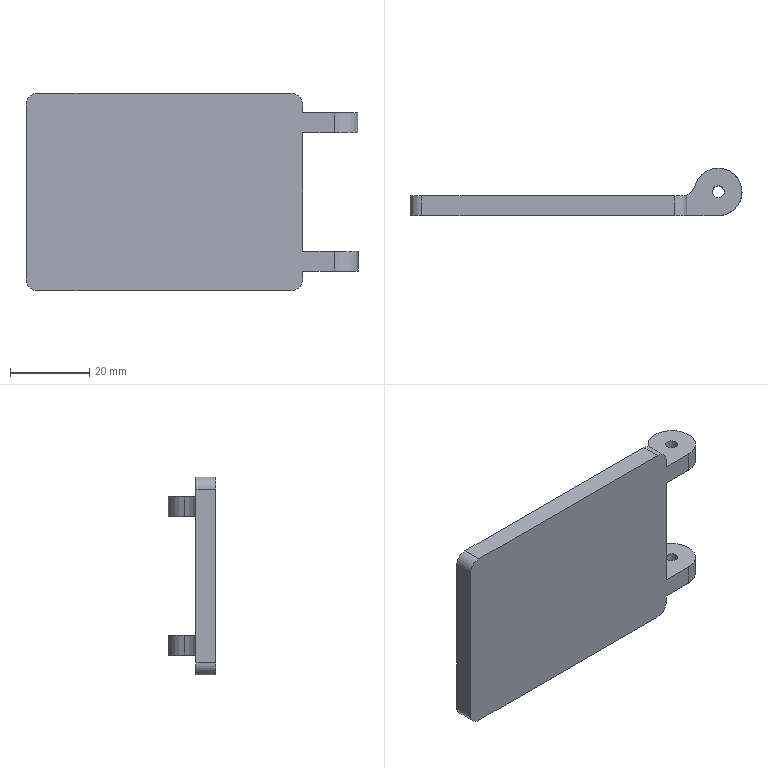Component | SolidWorks | 22FuelTankCap-1 | 1 solid | 25 faces | box 84 x 12 x 50 mm | volume 18718 mm3 | cylinder 13 | plane 12 | commonest cylinder face diameters 12 x5 3 x4 6 x4
STEP:
#1=CARTESIAN_POINT('',(3.204,14.835,19.37));
#2=VERTEX_POINT('',#1);
#3=CARTESIAN_POINT('',(3.322,14.835,19.37));
#4=VERTEX_POINT('',#3);
#5=CARTESIAN_POINT('',(3.263,14.835,19.37));
#6=DIRECTION('',(0.,0.,1.));
#7=DIRECTION('',(1.,0.,0.));
#8=AXIS2_PLACEMENT_3D('',#5,#6,#7);
#9=CIRCLE('',#8,0.05906);
#10=EDGE_CURVE('',#2,#4,#9,.T.);
#11=ORIENTED_EDGE('',*,*,#10,.F.);
#12=CARTESIAN_POINT('',(3.204,14.835,19.567));
#13=VERTEX_POINT('',#12);
#14=CARTESIAN_POINT('',(3.204,14.835,19.37));
#15=DIRECTION('',(0.,0.,1.));
#16=VECTOR('',#15,39.37);
#17=LINE('',#14,#16);
#18=EDGE_CURVE('',#2,#13,#17,.T.);
#19=ORIENTED_EDGE('',*,*,#18,.T.);
#20=CARTESIAN_POINT('',(3.322,14.835,19.567));
#21=VERTEX_POINT('',#20);
#22=CARTESIAN_POINT('',(3.263,14.835,19.567));
#23=DIRECTION('',(0.,0.,1.));
#24=DIRECTION('',(1.,0.,0.));
#25=AXIS2_PLACEMENT_3D('',#22,#23,#24);
#26=CIRCLE('',#25,0.05906);
#27=EDGE_CURVE('',#13,#21,#26,.T.);
#28=ORIENTED_EDGE('',*,*,#27,.T.);
#29=CARTESIAN_POINT('',(3.322,14.835,19.37));
#30=DIRECTION('',(0.,0.,1.));
#31=VECTOR('',#30,39.37);
#32=LINE('',#29,#31);
#33=EDGE_CURVE('',#4,#21,#32,.T.);
#34=ORIENTED_EDGE('',*,*,#33,.F.);
#35=EDGE_LOOP('',(#11,#19,#28,#34));
#36=FACE_OUTER_BOUND('',#35,.T.);
#37=CARTESIAN_POINT('',(3.263,14.835,19.37));
#38=DIRECTION('',(0.,0.,1.));
#39=DIRECTION('',(1.,0.,0.));
#40=AXIS2_PLACEMENT_3D('',#37,#38,#39);
#41=CYLINDRICAL_SURFACE('',#40,0.05906);
#42=ADVANCED_FACE('',(#36),#41,.F.);
#43=CARTESIAN_POINT('',(3.263,14.599,19.37));
#44=VERTEX_POINT('',#43);
#45=CARTESIAN_POINT('',(3.499,14.835,19.37));
#46=VERTEX_POINT('',#45);
#47=CARTESIAN_POINT('',(3.263,14.835,19.37));
#48=DIRECTION('',(0.,0.,1.));
#49=DIRECTION('',(1.,0.,0.));
#50=AXIS2_PLACEMENT_3D('',#47,#48,#49);
#51=CIRCLE('',#50,0.2362);
#52=EDGE_CURVE('',#44,#46,#51,.T.);
#53=ORIENTED_EDGE('',*,*,#52,.T.);
#54=CARTESIAN_POINT('',(3.499,14.835,19.567));
#55=VERTEX_POINT('',#54);
#56=CARTESIAN_POINT('',(3.499,14.835,19.37));
#57=DIRECTION('',(0.,0.,1.));
#58=VECTOR('',#57,39.37);
#59=LINE('',#56,#58);
#60=EDGE_CURVE('',#46,#55,#59,.T.);
#61=ORIENTED_EDGE('',*,*,#60,.T.);
#62=CARTESIAN_POINT('',(3.263,14.599,19.567));
#63=VERTEX_POINT('',#62);
#64=CARTESIAN_POINT('',(3.263,14.835,19.567));
#65=DIRECTION('',(0.,0.,1.));
#66=DIRECTION('',(1.,0.,0.));
#67=AXIS2_PLACEMENT_3D('',#64,#65,#66);
#68=CIRCLE('',#67,0.2362);
#69=EDGE_CURVE('',#63,#55,#68,.T.);
#70=ORIENTED_EDGE('',*,*,#69,.F.);
#71=CARTESIAN_POINT('',(3.263,14.599,19.37));
#72=DIRECTION('',(0.,0.,1.));
#73=VECTOR('',#72,39.37);
#74=LINE('',#71,#73);
#75=EDGE_CURVE('',#44,#63,#74,.T.);
#76=ORIENTED_EDGE('',*,*,#75,.F.);
#77=EDGE_LOOP('',(#53,#61,#70,#76));
#78=FACE_OUTER_BOUND('',#77,.T.);
#79=CARTESIAN_POINT('',(3.263,14.835,19.37));
#80=DIRECTION('',(0.,0.,1.));
#81=DIRECTION('',(1.,0.,0.));
#82=AXIS2_PLACEMENT_3D('',#79,#80,#81);
#83=CYLINDRICAL_SURFACE('',#82,0.2362);
#84=ADVANCED_FACE('',(#78),#83,.T.);
#85=CARTESIAN_POINT('',(3.204,14.835,20.945));
#86=VERTEX_POINT('',#85);
#87=CARTESIAN_POINT('',(3.322,14.835,20.945));
#88=VERTEX_POINT('',#87);
#89=CARTESIAN_POINT('',(3.263,14.835,20.945));
#90=DIRECTION('',(0.,0.,1.));
#91=DIRECTION('',(1.,0.,0.));
#92=AXIS2_PLACEMENT_3D('',#89,#90,#91);
#93=CIRCLE('',#92,0.05906);
#94=EDGE_CURVE('',#86,#88,#93,.T.);
#95=ORIENTED_EDGE('',*,*,#94,.T.);
#96=CARTESIAN_POINT('',(3.322,14.835,20.748));
#97=VERTEX_POINT('',#96);
#98=CARTESIAN_POINT('',(3.322,14.835,20.945));
#99=DIRECTION('',(0.,0.,-1.));
#100=VECTOR('',#99,39.37);
#101=LINE('',#98,#100);
#102=EDGE_CURVE('',#88,#97,#101,.T.);
#103=ORIENTED_EDGE('',*,*,#102,.T.);
#104=CARTESIAN_POINT('',(3.204,14.835,20.748));
#105=VERTEX_POINT('',#104);
#106=CARTESIAN_POINT('',(3.263,14.835,20.748));
#107=DIRECTION('',(0.,0.,1.));
#108=DIRECTION('',(1.,0.,0.));
#109=AXIS2_PLACEMENT_3D('',#106,#107,#108);
#110=CIRCLE('',#109,0.05906);
#111=EDGE_CURVE('',#105,#97,#110,.T.);
#112=ORIENTED_EDGE('',*,*,#111,.F.);
#113=CARTESIAN_POINT('',(3.204,14.835,20.945));
#114=DIRECTION('',(0.,0.,-1.));
#115=VECTOR('',#114,39.37);
#116=LINE('',#113,#115);
#117=EDGE_CURVE('',#86,#105,#116,.T.);
#118=ORIENTED_EDGE('',*,*,#117,.F.);
#119=EDGE_LOOP('',(#95,#103,#112,#118));
#120=FACE_OUTER_BOUND('',#119,.T.);
#121=CARTESIAN_POINT('',(3.263,14.835,20.945));
#122=DIRECTION('',(0.,0.,-1.));
#123=DIRECTION('',(-1.,0.,0.));
#124=AXIS2_PLACEMENT_3D('',#121,#122,#123);
#125=CYLINDRICAL_SURFACE('',#124,0.05906);
#126=ADVANCED_FACE('',(#120),#125,.F.);
#127=CARTESIAN_POINT('',(2.948,14.796,19.567));
#128=VERTEX_POINT('',#127);
#129=CARTESIAN_POINT('',(2.948,14.599,19.567));
#130=VERTEX_POINT('',#129);
#131=CARTESIAN_POINT('',(2.948,14.599,19.567));
#132=DIRECTION('',(0.,-1.,0.));
#133=VECTOR('',#132,39.37);
#134=LINE('',#131,#133);
#135=EDGE_CURVE('',#128,#130,#134,.T.);
#136=ORIENTED_EDGE('',*,*,#135,.F.);
#137=CARTESIAN_POINT('',(2.948,14.796,20.748));
#138=VERTEX_POINT('',#137);
#139=CARTESIAN_POINT('',(2.948,14.796,19.291));
#140=DIRECTION('',(0.,0.,-1.));
#141=VECTOR('',#140,39.37);
#142=LINE('',#139,#141);
#143=EDGE_CURVE('',#138,#128,#142,.T.);
#144=ORIENTED_EDGE('',*,*,#143,.F.);
#145=CARTESIAN_POINT('',(2.948,14.599,20.748));
#146=VERTEX_POINT('',#145);
#147=CARTESIAN_POINT('',(2.948,14.599,20.748));
#148=DIRECTION('',(0.,-1.,0.));
#149=VECTOR('',#148,39.37);
#150=LINE('',#147,#149);
#151=EDGE_CURVE('',#138,#146,#150,.T.);
#152=ORIENTED_EDGE('',*,*,#151,.T.);
#153=CARTESIAN_POINT('',(2.948,14.599,19.291));
#154=DIRECTION('',(0.,0.,-1.));
#155=VECTOR('',#154,39.37);
#156=LINE('',#153,#155);
#157=EDGE_CURVE('',#146,#130,#156,.T.);
#158=ORIENTED_EDGE('',*,*,#157,.T.);
#159=EDGE_LOOP('',(#136,#144,#152,#158));
#160=FACE_OUTER_BOUND('',#159,.T.);
#161=CARTESIAN_POINT('',(2.948,14.796,19.291));
#162=DIRECTION('',(-1.,0.,0.));
#163=DIRECTION('',(0.,0.,1.));
#164=AXIS2_PLACEMENT_3D('',#161,#162,#163);
#165=PLANE('',#164);
#166=ADVANCED_FACE('',(#160),#165,.F.);
#167=CARTESIAN_POINT('',(2.948,14.796,19.37));
#168=VERTEX_POINT('',#167);
#169=CARTESIAN_POINT('',(2.948,14.796,19.291));
#170=VERTEX_POINT('',#169);
#171=CARTESIAN_POINT('',(2.948,14.796,19.291));
#172=DIRECTION('',(0.,0.,-1.));
#173=VECTOR('',#172,39.37);
#174=LINE('',#171,#173);
#175=EDGE_CURVE('',#168,#170,#174,.T.);
#176=ORIENTED_EDGE('',*,*,#175,.F.);
#177=CARTESIAN_POINT('',(2.948,14.599,19.37));
#178=VERTEX_POINT('',#177);
#179=CARTESIAN_POINT('',(2.948,14.599,19.37));
#180=DIRECTION('',(0.,-1.,0.));
#181=VECTOR('',#180,39.37);
#182=LINE('',#179,#181);
#183=EDGE_CURVE('',#168,#178,#182,.T.);
#184=ORIENTED_EDGE('',*,*,#183,.T.);
#185=CARTESIAN_POINT('',(2.948,14.599,19.291));
#186=VERTEX_POINT('',#185);
#187=CARTESIAN_POINT('',(2.948,14.599,19.291));
#188=DIRECTION('',(0.,0.,-1.));
#189=VECTOR('',#188,39.37);
#190=LINE('',#187,#189);
#191=EDGE_CURVE('',#178,#186,#190,.T.);
#192=ORIENTED_EDGE('',*,*,#191,.T.);
#193=CARTESIAN_POINT('',(2.948,14.796,19.291));
#194=DIRECTION('',(0.,-1.,0.));
#195=VECTOR('',#194,39.37);
#196=LINE('',#193,#195);
#197=EDGE_CURVE('',#170,#186,#196,.T.);
#198=ORIENTED_EDGE('',*,*,#197,.F.);
#199=EDGE_LOOP('',(#176,#184,#192,#198));
#200=FACE_OUTER_BOUND('',#199,.T.);
#201=CARTESIAN_POINT('',(2.948,14.796,19.291));
#202=DIRECTION('',(-1.,0.,0.));
#203=DIRECTION('',(0.,0.,1.));
#204=AXIS2_PLACEMENT_3D('',#201,#202,#203);
#205=PLANE('',#204);
#206=ADVANCED_FACE('',(#200),#205,.F.);
#207=CARTESIAN_POINT('',(2.83,14.599,19.173));
#208=VERTEX_POINT('',#207);
#209=CARTESIAN_POINT('',(2.83,14.599,19.291));
#210=DIRECTION('',(0.,1.,0.));
#211=DIRECTION('',(0.,0.,-1.));
#212=AXIS2_PLACEMENT_3D('',#209,#210,#211);
#213=CIRCLE('',#212,0.1181);
#214=EDGE_CURVE('',#186,#208,#213,.T.);
#215=ORIENTED_EDGE('',*,*,#214,.T.);
#216=CARTESIAN_POINT('',(2.83,14.796,19.173));
#217=VERTEX_POINT('',#216);
#218=CARTESIAN_POINT('',(2.83,14.796,19.173));
#219=DIRECTION('',(0.,-1.,0.));
#220=VECTOR('',#219,39.37);
#221=LINE('',#218,#220);
#222=EDGE_CURVE('',#217,#208,#221,.T.);
#223=ORIENTED_EDGE('',*,*,#222,.F.);
#224=CARTESIAN_POINT('',(2.83,14.796,19.291));
#225=DIRECTION('',(0.,1.,0.));
#226=DIRECTION('',(0.,0.,-1.));
#227=AXIS2_PLACEMENT_3D('',#224,#225,#226);
#228=CIRCLE('',#227,0.1181);
#229=EDGE_CURVE('',#170,#217,#228,.T.);
#230=ORIENTED_EDGE('',*,*,#229,.F.);
#231=ORIENTED_EDGE('',*,*,#197,.T.);
#232=EDGE_LOOP('',(#215,#223,#230,#231));
#233=FACE_OUTER_BOUND('',#232,.T.);
#234=CARTESIAN_POINT('',(2.83,14.796,19.291));
#235=DIRECTION('',(0.,-1.,0.));
#236=DIRECTION('',(0.,0.,-1.));
#237=AXIS2_PLACEMENT_3D('',#234,#235,#236);
#238=CYLINDRICAL_SURFACE('',#237,0.1181);
#239=ADVANCED_FACE('',(#233),#238,.T.);
#240=CARTESIAN_POINT('',(0.3104,14.599,19.173));
#241=VERTEX_POINT('',#240);
#242=CARTESIAN_POINT('',(0.3104,14.599,19.173));
#243=DIRECTION('',(-1.,0.,0.));
#244=VECTOR('',#243,39.37);
#245=LINE('',#242,#244);
#246=EDGE_CURVE('',#208,#241,#245,.T.);
#247=ORIENTED_EDGE('',*,*,#246,.T.);
#248=CARTESIAN_POINT('',(0.3104,14.796,19.173));
#249=VERTEX_POINT('',#248);
#250=CARTESIAN_POINT('',(0.3104,14.796,19.173));
#251=DIRECTION('',(0.,-1.,0.));
#252=VECTOR('',#251,39.37);
#253=LINE('',#250,#252);
#254=EDGE_CURVE('',#249,#241,#253,.T.);
#255=ORIENTED_EDGE('',*,*,#254,.F.);
#256=CARTESIAN_POINT('',(0.3104,14.796,19.173));
#257=DIRECTION('',(-1.,0.,0.));
#258=VECTOR('',#257,39.37);
#259=LINE('',#256,#258);
#260=EDGE_CURVE('',#217,#249,#259,.T.);
#261=ORIENTED_EDGE('',*,*,#260,.F.);
#262=ORIENTED_EDGE('',*,*,#222,.T.);
#263=EDGE_LOOP('',(#247,#255,#261,#262));
#264=FACE_OUTER_BOUND('',#263,.T.);
#265=CARTESIAN_POINT('',(0.3104,14.796,19.173));
#266=DIRECTION('',(0.,0.,1.));
#267=DIRECTION('',(1.,0.,0.));
#268=AXIS2_PLACEMENT_3D('',#265,#266,#267);
#269=PLANE('',#268);
#270=ADVANCED_FACE('',(#264),#269,.F.);
#271=CARTESIAN_POINT('',(0.1923,14.599,19.291));
#272=VERTEX_POINT('',#271);
#273=CARTESIAN_POINT('',(0.3104,14.599,19.291));
#274=DIRECTION('',(0.,1.,0.));
#275=DIRECTION('',(0.,0.,1.));
#276=AXIS2_PLACEMENT_3D('',#273,#274,#275);
#277=CIRCLE('',#276,0.1181);
#278=EDGE_CURVE('',#241,#272,#277,.T.);
#279=ORIENTED_EDGE('',*,*,#278,.T.);
#280=CARTESIAN_POINT('',(0.1923,14.796,19.291));
#281=VERTEX_POINT('',#280);
#282=CARTESIAN_POINT('',(0.1923,14.796,19.291));
#283=DIRECTION('',(0.,-1.,0.));
#284=VECTOR('',#283,39.37);
#285=LINE('',#282,#284);
#286=EDGE_CURVE('',#281,#272,#285,.T.);
#287=ORIENTED_EDGE('',*,*,#286,.F.);
#288=CARTESIAN_POINT('',(0.3104,14.796,19.291));
#289=DIRECTION('',(0.,1.,0.));
#290=DIRECTION('',(0.,0.,1.));
#291=AXIS2_PLACEMENT_3D('',#288,#289,#290);
#292=CIRCLE('',#291,0.1181);
#293=EDGE_CURVE('',#249,#281,#292,.T.);
#294=ORIENTED_EDGE('',*,*,#293,.F.);
#295=ORIENTED_EDGE('',*,*,#254,.T.);
#296=EDGE_LOOP('',(#279,#287,#294,#295));
#297=FACE_OUTER_BOUND('',#296,.T.);
#298=CARTESIAN_POINT('',(0.3104,14.796,19.291));
#299=DIRECTION('',(0.,-1.,0.));
#300=DIRECTION('',(0.,0.,-1.));
#301=AXIS2_PLACEMENT_3D('',#298,#299,#300);
#302=CYLINDRICAL_SURFACE('',#301,0.1181);
#303=ADVANCED_FACE('',(#297),#302,.T.);
#304=CARTESIAN_POINT('',(0.1923,14.599,21.024));
#305=VERTEX_POINT('',#304);
#306=CARTESIAN_POINT('',(0.1923,14.599,19.291));
#307=DIRECTION('',(0.,0.,1.));
#308=VECTOR('',#307,39.37);
#309=LINE('',#306,#308);
#310=EDGE_CURVE('',#272,#305,#309,.T.);
#311=ORIENTED_EDGE('',*,*,#310,.T.);
#312=CARTESIAN_POINT('',(0.1923,14.796,21.024));
#313=VERTEX_POINT('',#312);
#314=CARTESIAN_POINT('',(0.1923,14.796,21.024));
#315=DIRECTION('',(0.,-1.,0.));
#316=VECTOR('',#315,39.37);
#317=LINE('',#314,#316);
#318=EDGE_CURVE('',#313,#305,#317,.T.);
#319=ORIENTED_EDGE('',*,*,#318,.F.);
#320=CARTESIAN_POINT('',(0.1923,14.796,19.291));
#321=DIRECTION('',(0.,0.,1.));
#322=VECTOR('',#321,39.37);
#323=LINE('',#320,#322);
#324=EDGE_CURVE('',#281,#313,#323,.T.);
#325=ORIENTED_EDGE('',*,*,#324,.F.);
#326=ORIENTED_EDGE('',*,*,#286,.T.);
#327=EDGE_LOOP('',(#311,#319,#325,#326));
#328=FACE_OUTER_BOUND('',#327,.T.);
#329=CARTESIAN_POINT('',(0.1923,14.796,19.291));
#330=DIRECTION('',(1.,0.,0.));
#331=DIRECTION('',(0.,0.,-1.));
#332=AXIS2_PLACEMENT_3D('',#329,#330,#331);
#333=PLANE('',#332);
#334=ADVANCED_FACE('',(#328),#333,.F.);
#335=CARTESIAN_POINT('',(0.3104,14.599,21.142));
#336=VERTEX_POINT('',#335);
#337=CARTESIAN_POINT('',(0.3104,14.599,21.024));
#338=DIRECTION('',(0.,1.,0.));
#339=DIRECTION('',(0.,0.,1.));
#340=AXIS2_PLACEMENT_3D('',#337,#338,#339);
#341=CIRCLE('',#340,0.1181);
#342=EDGE_CURVE('',#305,#336,#341,.T.);
#343=ORIENTED_EDGE('',*,*,#342,.T.);
#344=CARTESIAN_POINT('',(0.3104,14.796,21.142));
#345=VERTEX_POINT('',#344);
#346=CARTESIAN_POINT('',(0.3104,14.796,21.142));
#347=DIRECTION('',(0.,-1.,0.));
#348=VECTOR('',#347,39.37);
#349=LINE('',#346,#348);
#350=EDGE_CURVE('',#345,#336,#349,.T.);
#351=ORIENTED_EDGE('',*,*,#350,.F.);
#352=CARTESIAN_POINT('',(0.3104,14.796,21.024));
#353=DIRECTION('',(0.,1.,0.));
#354=DIRECTION('',(0.,0.,1.));
#355=AXIS2_PLACEMENT_3D('',#352,#353,#354);
#356=CIRCLE('',#355,0.1181);
#357=EDGE_CURVE('',#313,#345,#356,.T.);
#358=ORIENTED_EDGE('',*,*,#357,.F.);
#359=ORIENTED_EDGE('',*,*,#318,.T.);
#360=EDGE_LOOP('',(#343,#351,#358,#359));
#361=FACE_OUTER_BOUND('',#360,.T.);
#362=CARTESIAN_POINT('',(0.3104,14.796,21.024));
#363=DIRECTION('',(0.,-1.,0.));
#364=DIRECTION('',(0.,0.,-1.));
#365=AXIS2_PLACEMENT_3D('',#362,#363,#364);
#366=CYLINDRICAL_SURFACE('',#365,0.1181);
#367=ADVANCED_FACE('',(#361),#366,.T.);
#368=CARTESIAN_POINT('',(2.83,14.599,21.142));
#369=VERTEX_POINT('',#368);
#370=CARTESIAN_POINT('',(0.3104,14.599,21.142));
#371=DIRECTION('',(1.,0.,0.));
#372=VECTOR('',#371,39.37);
#373=LINE('',#370,#372);
#374=EDGE_CURVE('',#336,#369,#373,.T.);
#375=ORIENTED_EDGE('',*,*,#374,.T.);
#376=CARTESIAN_POINT('',(2.83,14.796,21.142));
#377=VERTEX_POINT('',#376);
#378=CARTESIAN_POINT('',(2.83,14.796,21.142));
#379=DIRECTION('',(0.,-1.,0.));
#380=VECTOR('',#379,39.37);
#381=LINE('',#378,#380);
#382=EDGE_CURVE('',#377,#369,#381,.T.);
#383=ORIENTED_EDGE('',*,*,#382,.F.);
#384=CARTESIAN_POINT('',(0.3104,14.796,21.142));
#385=DIRECTION('',(1.,0.,0.));
#386=VECTOR('',#385,39.37);
#387=LINE('',#384,#386);
#388=EDGE_CURVE('',#345,#377,#387,.T.);
#389=ORIENTED_EDGE('',*,*,#388,.F.);
#390=ORIENTED_EDGE('',*,*,#350,.T.);
#391=EDGE_LOOP('',(#375,#383,#389,#390));
#392=FACE_OUTER_BOUND('',#391,.T.);
#393=CARTESIAN_POINT('',(0.3104,14.796,21.142));
#394=DIRECTION('',(0.,0.,-1.));
#395=DIRECTION('',(-1.,0.,0.));
#396=AXIS2_PLACEMENT_3D('',#393,#394,#395);
#397=PLANE('',#396);
#398=ADVANCED_FACE('',(#392),#397,.F.);
#399=CARTESIAN_POINT('',(2.948,14.599,21.024));
#400=VERTEX_POINT('',#399);
#401=CARTESIAN_POINT('',(2.83,14.599,21.024));
#402=DIRECTION('',(0.,1.,0.));
#403=DIRECTION('',(0.,0.,1.));
#404=AXIS2_PLACEMENT_3D('',#401,#402,#403);
#405=CIRCLE('',#404,0.1181);
#406=EDGE_CURVE('',#369,#400,#405,.T.);
#407=ORIENTED_EDGE('',*,*,#406,.T.);
#408=CARTESIAN_POINT('',(2.948,14.796,21.024));
#409=VERTEX_POINT('',#408);
#410=CARTESIAN_POINT('',(2.948,14.796,21.024));
#411=DIRECTION('',(0.,-1.,0.));
#412=VECTOR('',#411,39.37);
#413=LINE('',#410,#412);
#414=EDGE_CURVE('',#409,#400,#413,.T.);
#415=ORIENTED_EDGE('',*,*,#414,.F.);
#416=CARTESIAN_POINT('',(2.83,14.796,21.024));
#417=DIRECTION('',(0.,1.,0.));
#418=DIRECTION('',(0.,0.,1.));
#419=AXIS2_PLACEMENT_3D('',#416,#417,#418);
#420=CIRCLE('',#419,0.1181);
#421=EDGE_CURVE('',#377,#409,#420,.T.);
#422=ORIENTED_EDGE('',*,*,#421,.F.);
#423=ORIENTED_EDGE('',*,*,#382,.T.);
#424=EDGE_LOOP('',(#407,#415,#422,#423));
#425=FACE_OUTER_BOUND('',#424,.T.);
#426=CARTESIAN_POINT('',(2.83,14.796,21.024));
#427=DIRECTION('',(0.,-1.,0.));
#428=DIRECTION('',(0.,0.,-1.));
#429=AXIS2_PLACEMENT_3D('',#426,#427,#428);
#430=CYLINDRICAL_SURFACE('',#429,0.1181);
#431=ADVANCED_FACE('',(#425),#430,.T.);
#432=CARTESIAN_POINT('',(2.948,14.599,20.945));
#433=VERTEX_POINT('',#432);
#434=CARTESIAN_POINT('',(2.948,14.599,19.291));
#435=DIRECTION('',(0.,0.,-1.));
#436=VECTOR('',#435,39.37);
#437=LINE('',#434,#436);
#438=EDGE_CURVE('',#400,#433,#437,.T.);
#439=ORIENTED_EDGE('',*,*,#438,.T.);
#440=CARTESIAN_POINT('',(2.948,14.796,20.945));
#441=VERTEX_POINT('',#440);
#442=CARTESIAN_POINT('',(2.948,14.599,20.945));
#443=DIRECTION('',(0.,-1.,0.));
#444=VECTOR('',#443,39.37);
#445=LINE('',#442,#444);
#446=EDGE_CURVE('',#441,#433,#445,.T.);
#447=ORIENTED_EDGE('',*,*,#446,.F.);
#448=CARTESIAN_POINT('',(2.948,14.796,19.291));
#449=DIRECTION('',(0.,0.,-1.));
#450=VECTOR('',#449,39.37);
#451=LINE('',#448,#450);
#452=EDGE_CURVE('',#409,#441,#451,.T.);
#453=ORIENTED_EDGE('',*,*,#452,.F.);
#454=ORIENTED_EDGE('',*,*,#414,.T.);
#455=EDGE_LOOP('',(#439,#447,#453,#454));
#456=FACE_OUTER_BOUND('',#455,.T.);
#457=CARTESIAN_POINT('',(2.948,14.796,19.291));
#458=DIRECTION('',(-1.,0.,0.));
#459=DIRECTION('',(0.,0.,1.));
#460=AXIS2_PLACEMENT_3D('',#457,#458,#459);
#461=PLANE('',#460);
#462=ADVANCED_FACE('',(#456),#461,.F.);
#463=ORIENTED_EDGE('',*,*,#229,.T.);
#464=ORIENTED_EDGE('',*,*,#260,.T.);
#465=ORIENTED_EDGE('',*,*,#293,.T.);
#466=ORIENTED_EDGE('',*,*,#324,.T.);
#467=ORIENTED_EDGE('',*,*,#357,.T.);
#468=ORIENTED_EDGE('',*,*,#388,.T.);
#469=ORIENTED_EDGE('',*,*,#421,.T.);
#470=ORIENTED_EDGE('',*,*,#452,.T.);
#471=CARTESIAN_POINT('',(2.948,14.796,20.945));
#472=DIRECTION('',(0.,0.,-1.));
#473=VECTOR('',#472,39.37);
#474=LINE('',#471,#473);
#475=EDGE_CURVE('',#441,#138,#474,.T.);
#476=ORIENTED_EDGE('',*,*,#475,.T.);
#477=ORIENTED_EDGE('',*,*,#143,.T.);
#478=CARTESIAN_POINT('',(2.948,14.796,19.37));
#479=DIRECTION('',(0.,0.,1.));
#480=VECTOR('',#479,39.37);
#481=LINE('',#478,#480);
#482=EDGE_CURVE('',#168,#128,#481,.T.);
#483=ORIENTED_EDGE('',*,*,#482,.F.);
#484=ORIENTED_EDGE('',*,*,#175,.T.);
#485=EDGE_LOOP('',(#463,#464,#465,#466,#467,#468,#469,#470,#476,#477,#483,#484));
#486=FACE_OUTER_BOUND('',#485,.T.);
#487=CARTESIAN_POINT('',(2.83,14.796,19.291));
#488=DIRECTION('',(0.,-1.,0.));
#489=DIRECTION('',(0.,0.,-1.));
#490=AXIS2_PLACEMENT_3D('',#487,#488,#489);
#491=PLANE('',#490);
#492=ADVANCED_FACE('',(#486),#491,.F.);
#493=ORIENTED_EDGE('',*,*,#214,.F.);
#494=ORIENTED_EDGE('',*,*,#191,.F.);
#495=CARTESIAN_POINT('',(1.57,14.599,19.37));
#496=DIRECTION('',(-1.,0.,0.));
#497=VECTOR('',#496,39.37);
#498=LINE('',#495,#497);
#499=EDGE_CURVE('',#44,#178,#498,.T.);
#500=ORIENTED_EDGE('',*,*,#499,.F.);
#501=ORIENTED_EDGE('',*,*,#75,.T.);
#502=CARTESIAN_POINT('',(1.57,14.599,19.567));
#503=DIRECTION('',(-1.,0.,0.));
#504=VECTOR('',#503,39.37);
#505=LINE('',#502,#504);
#506=EDGE_CURVE('',#63,#130,#505,.T.);
#507=ORIENTED_EDGE('',*,*,#506,.T.);
#508=ORIENTED_EDGE('',*,*,#157,.F.);
#509=CARTESIAN_POINT('',(3.263,14.599,20.748));
#510=VERTEX_POINT('',#509);
#511=CARTESIAN_POINT('',(1.57,14.599,20.748));
#512=DIRECTION('',(-1.,0.,0.));
#513=VECTOR('',#512,39.37);
#514=LINE('',#511,#513);
#515=EDGE_CURVE('',#510,#146,#514,.T.);
#516=ORIENTED_EDGE('',*,*,#515,.F.);
#517=CARTESIAN_POINT('',(3.263,14.599,20.945));
#518=VERTEX_POINT('',#517);
#519=CARTESIAN_POINT('',(3.263,14.599,20.945));
#520=DIRECTION('',(0.,0.,-1.));
#521=VECTOR('',#520,39.37);
#522=LINE('',#519,#521);
#523=EDGE_CURVE('',#518,#510,#522,.T.);
#524=ORIENTED_EDGE('',*,*,#523,.F.);
#525=CARTESIAN_POINT('',(1.57,14.599,20.945));
#526=DIRECTION('',(-1.,0.,0.));
#527=VECTOR('',#526,39.37);
#528=LINE('',#525,#527);
#529=EDGE_CURVE('',#518,#433,#528,.T.);
#530=ORIENTED_EDGE('',*,*,#529,.T.);
#531=ORIENTED_EDGE('',*,*,#438,.F.);
#532=ORIENTED_EDGE('',*,*,#406,.F.);
#533=ORIENTED_EDGE('',*,*,#374,.F.);
#534=ORIENTED_EDGE('',*,*,#342,.F.);
#535=ORIENTED_EDGE('',*,*,#310,.F.);
#536=ORIENTED_EDGE('',*,*,#278,.F.);
#537=ORIENTED_EDGE('',*,*,#246,.F.);
#538=EDGE_LOOP('',(#493,#494,#500,#501,#507,#508,#516,#524,#530,#531,#532,#533,#534,#535,#536,#537));
#539=FACE_OUTER_BOUND('',#538,.T.);
#540=CARTESIAN_POINT('',(2.83,14.599,19.291));
#541=DIRECTION('',(0.,-1.,0.));
#542=DIRECTION('',(0.,0.,-1.));
#543=AXIS2_PLACEMENT_3D('',#540,#541,#542);
#544=PLANE('',#543);
#545=ADVANCED_FACE('',(#539),#544,.T.);
#546=CARTESIAN_POINT('',(3.04,14.914,20.748));
#547=VERTEX_POINT('',#546);
#548=CARTESIAN_POINT('',(2.818,14.993,20.748));
#549=DIRECTION('',(0.,0.,1.));
#550=DIRECTION('',(1.,0.,0.));
#551=AXIS2_PLACEMENT_3D('',#548,#549,#550);
#552=CIRCLE('',#551,0.2362);
#553=EDGE_CURVE('',#138,#547,#552,.T.);
#554=ORIENTED_EDGE('',*,*,#553,.F.);
#555=ORIENTED_EDGE('',*,*,#475,.F.);
#556=CARTESIAN_POINT('',(3.04,14.914,20.945));
#557=VERTEX_POINT('',#556);
#558=CARTESIAN_POINT('',(2.818,14.993,20.945));
#559=DIRECTION('',(0.,0.,1.));
#560=DIRECTION('',(1.,0.,0.));
#561=AXIS2_PLACEMENT_3D('',#558,#559,#560);
#562=CIRCLE('',#561,0.2362);
#563=EDGE_CURVE('',#441,#557,#562,.T.);
#564=ORIENTED_EDGE('',*,*,#563,.T.);
#565=CARTESIAN_POINT('',(3.04,14.914,20.945));
#566=DIRECTION('',(0.,0.,-1.));
#567=VECTOR('',#566,39.37);
#568=LINE('',#565,#567);
#569=EDGE_CURVE('',#557,#547,#568,.T.);
#570=ORIENTED_EDGE('',*,*,#569,.T.);
#571=EDGE_LOOP('',(#554,#555,#564,#570));
#572=FACE_OUTER_BOUND('',#571,.T.);
#573=CARTESIAN_POINT('',(2.818,14.993,20.945));
#574=DIRECTION('',(0.,0.,-1.));
#575=DIRECTION('',(-1.,0.,0.));
#576=AXIS2_PLACEMENT_3D('',#573,#574,#575);
#577=CYLINDRICAL_SURFACE('',#576,0.2362);
#578=ADVANCED_FACE('',(#572),#577,.F.);
#579=CARTESIAN_POINT('',(3.263,14.835,20.748));
#580=DIRECTION('',(0.,0.,1.));
#581=DIRECTION('',(1.,0.,0.));
#582=AXIS2_PLACEMENT_3D('',#579,#580,#581);
#583=CIRCLE('',#582,0.2362);
#584=EDGE_CURVE('',#510,#547,#583,.T.);
#585=ORIENTED_EDGE('',*,*,#584,.T.);
#586=ORIENTED_EDGE('',*,*,#569,.F.);
#587=CARTESIAN_POINT('',(3.263,14.835,20.945));
#588=DIRECTION('',(0.,0.,1.));
#589=DIRECTION('',(1.,0.,0.));
#590=AXIS2_PLACEMENT_3D('',#587,#588,#589);
#591=CIRCLE('',#590,0.2362);
#592=EDGE_CURVE('',#518,#557,#591,.T.);
#593=ORIENTED_EDGE('',*,*,#592,.F.);
#594=ORIENTED_EDGE('',*,*,#523,.T.);
#595=EDGE_LOOP('',(#585,#586,#593,#594));
#596=FACE_OUTER_BOUND('',#595,.T.);
#597=CARTESIAN_POINT('',(3.263,14.835,20.945));
#598=DIRECTION('',(0.,0.,-1.));
#599=DIRECTION('',(-1.,0.,0.));
#600=AXIS2_PLACEMENT_3D('',#597,#598,#599);
#601=CYLINDRICAL_SURFACE('',#600,0.2362);
#602=ADVANCED_FACE('',(#596),#601,.T.);
#603=ORIENTED_EDGE('',*,*,#102,.F.);
#604=CARTESIAN_POINT('',(3.263,14.835,20.945));
#605=DIRECTION('',(0.,0.,1.));
#606=DIRECTION('',(1.,0.,0.));
#607=AXIS2_PLACEMENT_3D('',#604,#605,#606);
#608=CIRCLE('',#607,0.05906);
#609=EDGE_CURVE('',#88,#86,#608,.T.);
#610=ORIENTED_EDGE('',*,*,#609,.T.);
#611=ORIENTED_EDGE('',*,*,#117,.T.);
#612=CARTESIAN_POINT('',(3.263,14.835,20.748));
#613=DIRECTION('',(0.,0.,1.));
#614=DIRECTION('',(1.,0.,0.));
#615=AXIS2_PLACEMENT_3D('',#612,#613,#614);
#616=CIRCLE('',#615,0.05906);
#617=EDGE_CURVE('',#97,#105,#616,.T.);
#618=ORIENTED_EDGE('',*,*,#617,.F.);
#619=EDGE_LOOP('',(#603,#610,#611,#618));
#620=FACE_OUTER_BOUND('',#619,.T.);
#621=CARTESIAN_POINT('',(3.263,14.835,20.945));
#622=DIRECTION('',(0.,0.,-1.));
#623=DIRECTION('',(-1.,0.,0.));
#624=AXIS2_PLACEMENT_3D('',#621,#622,#623);
#625=CYLINDRICAL_SURFACE('',#624,0.05906);
#626=ADVANCED_FACE('',(#620),#625,.F.);
#627=ORIENTED_EDGE('',*,*,#563,.F.);
#628=ORIENTED_EDGE('',*,*,#446,.T.);
#629=ORIENTED_EDGE('',*,*,#529,.F.);
#630=ORIENTED_EDGE('',*,*,#592,.T.);
#631=EDGE_LOOP('',(#627,#628,#629,#630));
#632=FACE_OUTER_BOUND('',#631,.T.);
#633=ORIENTED_EDGE('',*,*,#94,.F.);
#634=ORIENTED_EDGE('',*,*,#609,.F.);
#635=EDGE_LOOP('',(#633,#634));
#636=FACE_BOUND('',#635,.T.);
#637=CARTESIAN_POINT('',(1.57,14.599,20.945));
#638=DIRECTION('',(0.,0.,1.));
#639=DIRECTION('',(1.,0.,0.));
#640=AXIS2_PLACEMENT_3D('',#637,#638,#639);
#641=PLANE('',#640);
#642=ADVANCED_FACE('',(#632,#636),#641,.T.);
#643=ORIENTED_EDGE('',*,*,#553,.T.);
#644=ORIENTED_EDGE('',*,*,#584,.F.);
#645=ORIENTED_EDGE('',*,*,#515,.T.);
#646=ORIENTED_EDGE('',*,*,#151,.F.);
#647=EDGE_LOOP('',(#643,#644,#645,#646));
#648=FACE_OUTER_BOUND('',#647,.T.);
#649=ORIENTED_EDGE('',*,*,#111,.T.);
#650=ORIENTED_EDGE('',*,*,#617,.T.);
#651=EDGE_LOOP('',(#649,#650));
#652=FACE_BOUND('',#651,.T.);
#653=CARTESIAN_POINT('',(1.57,14.599,20.748));
#654=DIRECTION('',(0.,0.,1.));
#655=DIRECTION('',(1.,0.,0.));
#656=AXIS2_PLACEMENT_3D('',#653,#654,#655);
#657=PLANE('',#656);
#658=ADVANCED_FACE('',(#648,#652),#657,.F.);
#659=CARTESIAN_POINT('',(3.04,14.914,19.567));
#660=VERTEX_POINT('',#659);
#661=CARTESIAN_POINT('',(2.818,14.993,19.567));
#662=DIRECTION('',(0.,0.,1.));
#663=DIRECTION('',(1.,0.,0.));
#664=AXIS2_PLACEMENT_3D('',#661,#662,#663);
#665=CIRCLE('',#664,0.2362);
#666=EDGE_CURVE('',#128,#660,#665,.T.);
#667=ORIENTED_EDGE('',*,*,#666,.T.);
#668=CARTESIAN_POINT('',(3.04,14.914,19.37));
#669=VERTEX_POINT('',#668);
#670=CARTESIAN_POINT('',(3.04,14.914,19.37));
#671=DIRECTION('',(0.,0.,1.));
#672=VECTOR('',#671,39.37);
#673=LINE('',#670,#672);
#674=EDGE_CURVE('',#669,#660,#673,.T.);
#675=ORIENTED_EDGE('',*,*,#674,.F.);
#676=CARTESIAN_POINT('',(2.818,14.993,19.37));
#677=DIRECTION('',(0.,0.,1.));
#678=DIRECTION('',(1.,0.,0.));
#679=AXIS2_PLACEMENT_3D('',#676,#677,#678);
#680=CIRCLE('',#679,0.2362);
#681=EDGE_CURVE('',#168,#669,#680,.T.);
#682=ORIENTED_EDGE('',*,*,#681,.F.);
#683=ORIENTED_EDGE('',*,*,#482,.T.);
#684=EDGE_LOOP('',(#667,#675,#682,#683));
#685=FACE_OUTER_BOUND('',#684,.T.);
#686=CARTESIAN_POINT('',(2.818,14.993,19.37));
#687=DIRECTION('',(0.,0.,1.));
#688=DIRECTION('',(1.,0.,0.));
#689=AXIS2_PLACEMENT_3D('',#686,#687,#688);
#690=CYLINDRICAL_SURFACE('',#689,0.2362);
#691=ADVANCED_FACE('',(#685),#690,.F.);
#692=ORIENTED_EDGE('',*,*,#60,.F.);
#693=CARTESIAN_POINT('',(3.263,14.835,19.37));
#694=DIRECTION('',(0.,0.,1.));
#695=DIRECTION('',(1.,0.,0.));
#696=AXIS2_PLACEMENT_3D('',#693,#694,#695);
#697=CIRCLE('',#696,0.2362);
#698=EDGE_CURVE('',#46,#669,#697,.T.);
#699=ORIENTED_EDGE('',*,*,#698,.T.);
#700=ORIENTED_EDGE('',*,*,#674,.T.);
#701=CARTESIAN_POINT('',(3.263,14.835,19.567));
#702=DIRECTION('',(0.,0.,1.));
#703=DIRECTION('',(1.,0.,0.));
#704=AXIS2_PLACEMENT_3D('',#701,#702,#703);
#705=CIRCLE('',#704,0.2362);
#706=EDGE_CURVE('',#55,#660,#705,.T.);
#707=ORIENTED_EDGE('',*,*,#706,.F.);
#708=EDGE_LOOP('',(#692,#699,#700,#707));
#709=FACE_OUTER_BOUND('',#708,.T.);
#710=CARTESIAN_POINT('',(3.263,14.835,19.37));
#711=DIRECTION('',(0.,0.,1.));
#712=DIRECTION('',(1.,0.,0.));
#713=AXIS2_PLACEMENT_3D('',#710,#711,#712);
#714=CYLINDRICAL_SURFACE('',#713,0.2362);
#715=ADVANCED_FACE('',(#709),#714,.T.);
#716=ORIENTED_EDGE('',*,*,#18,.F.);
#717=CARTESIAN_POINT('',(3.263,14.835,19.37));
#718=DIRECTION('',(0.,0.,1.));
#719=DIRECTION('',(1.,0.,0.));
#720=AXIS2_PLACEMENT_3D('',#717,#718,#719);
#721=CIRCLE('',#720,0.05906);
#722=EDGE_CURVE('',#4,#2,#721,.T.);
#723=ORIENTED_EDGE('',*,*,#722,.F.);
#724=ORIENTED_EDGE('',*,*,#33,.T.);
#725=CARTESIAN_POINT('',(3.263,14.835,19.567));
#726=DIRECTION('',(0.,0.,1.));
#727=DIRECTION('',(1.,0.,0.));
#728=AXIS2_PLACEMENT_3D('',#725,#726,#727);
#729=CIRCLE('',#728,0.05906);
#730=EDGE_CURVE('',#21,#13,#729,.T.);
#731=ORIENTED_EDGE('',*,*,#730,.T.);
#732=EDGE_LOOP('',(#716,#723,#724,#731));
#733=FACE_OUTER_BOUND('',#732,.T.);
#734=CARTESIAN_POINT('',(3.263,14.835,19.37));
#735=DIRECTION('',(0.,0.,1.));
#736=DIRECTION('',(1.,0.,0.));
#737=AXIS2_PLACEMENT_3D('',#734,#735,#736);
#738=CYLINDRICAL_SURFACE('',#737,0.05906);
#739=ADVANCED_FACE('',(#733),#738,.F.);
#740=ORIENTED_EDGE('',*,*,#681,.T.);
#741=ORIENTED_EDGE('',*,*,#698,.F.);
#742=ORIENTED_EDGE('',*,*,#52,.F.);
#743=ORIENTED_EDGE('',*,*,#499,.T.);
#744=ORIENTED_EDGE('',*,*,#183,.F.);
#745=EDGE_LOOP('',(#740,#741,#742,#743,#744));
#746=FACE_OUTER_BOUND('',#745,.T.);
#747=ORIENTED_EDGE('',*,*,#722,.T.);
#748=ORIENTED_EDGE('',*,*,#10,.T.);
#749=EDGE_LOOP('',(#747,#748));
#750=FACE_BOUND('',#749,.T.);
#751=CARTESIAN_POINT('',(1.57,14.599,19.37));
#752=DIRECTION('',(0.,0.,-1.));
#753=DIRECTION('',(1.,0.,0.));
#754=AXIS2_PLACEMENT_3D('',#751,#752,#753);
#755=PLANE('',#754);
#756=ADVANCED_FACE('',(#746,#750),#755,.T.);
#757=ORIENTED_EDGE('',*,*,#666,.F.);
#758=ORIENTED_EDGE('',*,*,#135,.T.);
#759=ORIENTED_EDGE('',*,*,#506,.F.);
#760=ORIENTED_EDGE('',*,*,#69,.T.);
#761=ORIENTED_EDGE('',*,*,#706,.T.);
#762=EDGE_LOOP('',(#757,#758,#759,#760,#761));
#763=FACE_OUTER_BOUND('',#762,.T.);
#764=ORIENTED_EDGE('',*,*,#730,.F.);
#765=ORIENTED_EDGE('',*,*,#27,.F.);
#766=EDGE_LOOP('',(#764,#765));
#767=FACE_BOUND('',#766,.T.);
#768=CARTESIAN_POINT('',(1.57,14.599,19.567));
#769=DIRECTION('',(0.,0.,-1.));
#770=DIRECTION('',(1.,0.,0.));
#771=AXIS2_PLACEMENT_3D('',#768,#769,#770);
#772=PLANE('',#771);
#773=ADVANCED_FACE('',(#763,#767),#772,.F.);
#774=CLOSED_SHELL('',(#42,#84,#126,#166,#206,#239,#270,#303,#334,#367,#398,#431,#462,#492,#545,#578,#602,#626,#642,#658,#691,#715,#739,#756,#773));
#775=MANIFOLD_SOLID_BREP('',#774);
#776=CARTESIAN_POINT('',(0.,0.,0.));
#777=DIRECTION('',(0.,0.,1.));
#778=DIRECTION('',(1.,0.,0.));
#779=AXIS2_PLACEMENT_3D('',#776,#777,#778);
#780=(LENGTH_UNIT()NAMED_UNIT(*)SI_UNIT($,.METRE.));
#781=LENGTH_MEASURE_WITH_UNIT(LENGTH_MEASURE(0.0254),#780);
#782=DIMENSIONAL_EXPONENTS(1.,0.,0.,0.,0.,0.,0.);
#783=(CONVERSION_BASED_UNIT('',#781)LENGTH_UNIT()NAMED_UNIT(#782));
#784=UNCERTAINTY_MEASURE_WITH_UNIT(LENGTH_MEASURE(0.00001),#783,'','');
#785=(NAMED_UNIT(*)PLANE_ANGLE_UNIT()SI_UNIT($,.RADIAN.));
#786=(NAMED_UNIT(*)SI_UNIT($,.STERADIAN.)SOLID_ANGLE_UNIT());
#787=(GEOMETRIC_REPRESENTATION_CONTEXT(3)GLOBAL_UNCERTAINTY_ASSIGNED_CONTEXT((#784))GLOBAL_UNIT_ASSIGNED_CONTEXT((#783,#785,#786))REPRESENTATION_CONTEXT('',''));
#788=ADVANCED_BREP_SHAPE_REPRESENTATION('',(#775,#779),#787);
#789=COLOUR_RGB('',0.7922,0.8196,0.9333);
#790=FILL_AREA_STYLE_COLOUR('',#789);
#791=FILL_AREA_STYLE('',(#790));
#792=SURFACE_STYLE_FILL_AREA(#791);
#793=SURFACE_SIDE_STYLE('',(#792));
#794=SURFACE_STYLE_USAGE(.BOTH.,#793);
#795=PRESENTATION_STYLE_ASSIGNMENT((#794));
#796=STYLED_ITEM('',(#795),#775);
#797=(LENGTH_UNIT()NAMED_UNIT(*)SI_UNIT($,.METRE.));
#798=LENGTH_MEASURE_WITH_UNIT(LENGTH_MEASURE(0.0254),#797);
#799=DIMENSIONAL_EXPONENTS(1.,0.,0.,0.,0.,0.,0.);
#800=(CONVERSION_BASED_UNIT('',#798)LENGTH_UNIT()NAMED_UNIT(#799));
#801=UNCERTAINTY_MEASURE_WITH_UNIT(LENGTH_MEASURE(0.00001),#800,'','');
#802=(NAMED_UNIT(*)PLANE_ANGLE_UNIT()SI_UNIT($,.RADIAN.));
#803=(NAMED_UNIT(*)SI_UNIT($,.STERADIAN.)SOLID_ANGLE_UNIT());
#804=(GEOMETRIC_REPRESENTATION_CONTEXT(3)GLOBAL_UNCERTAINTY_ASSIGNED_CONTEXT((#801))GLOBAL_UNIT_ASSIGNED_CONTEXT((#800,#802,#803))REPRESENTATION_CONTEXT('',''));
#805=MECHANICAL_DESIGN_GEOMETRIC_PRESENTATION_REPRESENTATION('',(#796),#804);
#806=PRESENTATION_LAYER_ASSIGNMENT('','',(#796));